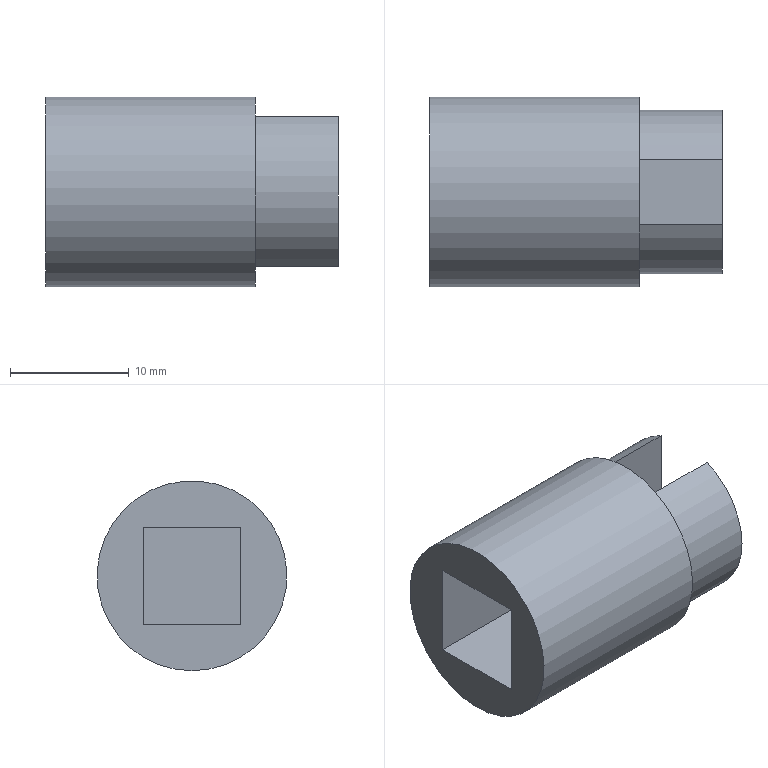Component | NX | SELECTOR_BLOCK | 1 solid | 17 faces | box 24.7 x 16 x 16 mm | volume 3205 mm3 | plane 14 | cylinder 3 | commonest cylinder face diameters 13.8 x2 16 x1
STEP:
#1=CARTESIAN_POINT('',(0.,0.,0.));
#2=DIRECTION('',(0.,0.,1.));
#3=DIRECTION('',(1.,0.,0.));
#4=AXIS2_PLACEMENT_3D('',#1,#2,#3);
#5=CARTESIAN_POINT('',(-16.538,-1.149,-12.417));
#6=VERTEX_POINT('',#5);
#7=CARTESIAN_POINT('',(-16.538,4.351,-12.417));
#8=VERTEX_POINT('',#7);
#9=CARTESIAN_POINT('',(-16.538,-1.149,-12.417));
#10=DIRECTION('',(0.,1.,-0.));
#11=VECTOR('',#10,1.);
#12=LINE('',#9,#11);
#13=CARTESIAN_POINT('',(-16.538,1.601,-11.667));
#14=DIRECTION('',(1.,0.,0.));
#15=DIRECTION('',(0.,0.,-1.));
#16=AXIS2_PLACEMENT_3D('',#13,#14,#15);
#17=PLANE('',#16);
#18=CARTESIAN_POINT('',(0.75,-2.75));
#19=DIRECTION('',(0.,1.));
#20=VECTOR('',#19,1.);
#21=LINE('',#18,#20);
#22=(GEOMETRIC_REPRESENTATION_CONTEXT(2)PARAMETRIC_REPRESENTATION_CONTEXT()REPRESENTATION_CONTEXT('',''));
#23=DEFINITIONAL_REPRESENTATION('',(#21),#22);
#24=PCURVE('',#17,#23);
#25=CARTESIAN_POINT('',(-23.538,-1.149,-12.417));
#26=DIRECTION('',(0.,-0.,-1.));
#27=DIRECTION('',(0.,1.,-0.));
#28=AXIS2_PLACEMENT_3D('',#25,#26,#27);
#29=PLANE('',#28);
#30=CARTESIAN_POINT('',(0.,7.));
#31=DIRECTION('',(1.,0.));
#32=VECTOR('',#31,1.);
#33=LINE('',#30,#32);
#34=(GEOMETRIC_REPRESENTATION_CONTEXT(2)PARAMETRIC_REPRESENTATION_CONTEXT()REPRESENTATION_CONTEXT('',''));
#35=DEFINITIONAL_REPRESENTATION('',(#33),#34);
#36=PCURVE('',#29,#35);
#37=SURFACE_CURVE('',#12,(#24,#36),.PCURVE_S1.);
#38=EDGE_CURVE('',#6,#8,#37,.T.);
#39=ORIENTED_EDGE('',*,*,#38,.T.);
#40=CARTESIAN_POINT('',(-16.538,4.351,-17.995));
#41=VERTEX_POINT('',#40);
#42=CARTESIAN_POINT('',(-16.538,4.351,-12.417));
#43=DIRECTION('',(0.,0.,-1.));
#44=VECTOR('',#43,1.);
#45=LINE('',#42,#44);
#46=CARTESIAN_POINT('',(0.75,2.75));
#47=DIRECTION('',(1.,0.));
#48=VECTOR('',#47,1.);
#49=LINE('',#46,#48);
#50=(GEOMETRIC_REPRESENTATION_CONTEXT(2)PARAMETRIC_REPRESENTATION_CONTEXT()REPRESENTATION_CONTEXT('',''));
#51=DEFINITIONAL_REPRESENTATION('',(#49),#50);
#52=PCURVE('',#17,#51);
#53=CARTESIAN_POINT('',(-23.538,4.351,-12.417));
#54=DIRECTION('',(0.,-1.,0.));
#55=DIRECTION('',(-1.,0.,0.));
#56=AXIS2_PLACEMENT_3D('',#53,#54,#55);
#57=PLANE('',#56);
#58=CARTESIAN_POINT('',(-7.,0.));
#59=DIRECTION('',(0.,1.));
#60=VECTOR('',#59,1.);
#61=LINE('',#58,#60);
#62=(GEOMETRIC_REPRESENTATION_CONTEXT(2)PARAMETRIC_REPRESENTATION_CONTEXT()REPRESENTATION_CONTEXT('',''));
#63=DEFINITIONAL_REPRESENTATION('',(#61),#62);
#64=PCURVE('',#57,#63);
#65=SURFACE_CURVE('',#45,(#52,#64),.PCURVE_S1.);
#66=EDGE_CURVE('',#8,#41,#65,.T.);
#67=ORIENTED_EDGE('',*,*,#66,.T.);
#68=CARTESIAN_POINT('',(-16.538,4.351,-5.338));
#69=VERTEX_POINT('',#68);
#70=CARTESIAN_POINT('',(-16.538,1.601,-11.667));
#71=DIRECTION('',(-1.,0.,0.));
#72=DIRECTION('',(0.,0.,-1.));
#73=AXIS2_PLACEMENT_3D('',#70,#71,#72);
#74=CIRCLE('',#73,6.9);
#75=CARTESIAN_POINT('',(6.9,0.));
#76=CARTESIAN_POINT('',(6.9,-11.951));
#77=CARTESIAN_POINT('',(-3.45,-5.976));
#78=CARTESIAN_POINT('',(-13.8,-0.));
#79=CARTESIAN_POINT('',(-3.45,5.976));
#80=CARTESIAN_POINT('',(6.9,11.951));
#81=CARTESIAN_POINT('',(6.9,0.));
#82=(BOUNDED_CURVE()B_SPLINE_CURVE(2,(#75,#76,#77,#78,#79,#80,#81),.UNSPECIFIED.,.T.,.F.)B_SPLINE_CURVE_WITH_KNOTS((1,2,2,2,2,1),(-2.094,0.,2.094,4.189,6.283,8.378),.UNSPECIFIED.)CURVE()GEOMETRIC_REPRESENTATION_ITEM()RATIONAL_B_SPLINE_CURVE((1.,0.5,1.,0.5,1.,0.5,1.))REPRESENTATION_ITEM(''));
#83=(GEOMETRIC_REPRESENTATION_CONTEXT(2)PARAMETRIC_REPRESENTATION_CONTEXT()REPRESENTATION_CONTEXT('',''));
#84=DEFINITIONAL_REPRESENTATION('',(#82),#83);
#85=PCURVE('',#17,#84);
#86=CARTESIAN_POINT('',(-23.538,1.601,-11.667));
#87=DIRECTION('',(1.,0.,0.));
#88=DIRECTION('',(0.,0.,-1.));
#89=AXIS2_PLACEMENT_3D('',#86,#87,#88);
#90=CYLINDRICAL_SURFACE('',#89,6.9);
#91=CARTESIAN_POINT('',(6.283,7.));
#92=DIRECTION('',(-1.,0.));
#93=VECTOR('',#92,1.);
#94=LINE('',#91,#93);
#95=(GEOMETRIC_REPRESENTATION_CONTEXT(2)PARAMETRIC_REPRESENTATION_CONTEXT()REPRESENTATION_CONTEXT('',''));
#96=DEFINITIONAL_REPRESENTATION('',(#94),#95);
#97=PCURVE('',#90,#96);
#98=SURFACE_CURVE('',#74,(#85,#97),.PCURVE_S1.);
#99=EDGE_CURVE('',#69,#41,#98,.T.);
#100=ORIENTED_EDGE('',*,*,#99,.F.);
#101=CARTESIAN_POINT('',(-16.538,4.351,-10.917));
#102=VERTEX_POINT('',#101);
#103=CARTESIAN_POINT('',(-16.538,4.351,-10.917));
#104=DIRECTION('',(0.,0.,1.));
#105=VECTOR('',#104,1.);
#106=LINE('',#103,#105);
#107=CARTESIAN_POINT('',(-0.75,2.75));
#108=DIRECTION('',(-1.,0.));
#109=VECTOR('',#108,1.);
#110=LINE('',#107,#109);
#111=(GEOMETRIC_REPRESENTATION_CONTEXT(2)PARAMETRIC_REPRESENTATION_CONTEXT()REPRESENTATION_CONTEXT('',''));
#112=DEFINITIONAL_REPRESENTATION('',(#110),#111);
#113=PCURVE('',#17,#112);
#114=CARTESIAN_POINT('',(-23.538,4.351,-10.917));
#115=DIRECTION('',(0.,1.,0.));
#116=DIRECTION('',(1.,0.,0.));
#117=AXIS2_PLACEMENT_3D('',#114,#115,#116);
#118=PLANE('',#117);
#119=CARTESIAN_POINT('',(7.,0.));
#120=DIRECTION('',(0.,-1.));
#121=VECTOR('',#120,1.);
#122=LINE('',#119,#121);
#123=(GEOMETRIC_REPRESENTATION_CONTEXT(2)PARAMETRIC_REPRESENTATION_CONTEXT()REPRESENTATION_CONTEXT('',''));
#124=DEFINITIONAL_REPRESENTATION('',(#122),#123);
#125=PCURVE('',#118,#124);
#126=SURFACE_CURVE('',#106,(#113,#125),.PCURVE_S1.);
#127=EDGE_CURVE('',#102,#69,#126,.T.);
#128=ORIENTED_EDGE('',*,*,#127,.F.);
#129=CARTESIAN_POINT('',(-16.538,-1.149,-10.917));
#130=VERTEX_POINT('',#129);
#131=CARTESIAN_POINT('',(-16.538,-1.149,-10.917));
#132=DIRECTION('',(0.,1.,0.));
#133=VECTOR('',#132,1.);
#134=LINE('',#131,#133);
#135=CARTESIAN_POINT('',(-0.75,-2.75));
#136=DIRECTION('',(-0.,1.));
#137=VECTOR('',#136,1.);
#138=LINE('',#135,#137);
#139=(GEOMETRIC_REPRESENTATION_CONTEXT(2)PARAMETRIC_REPRESENTATION_CONTEXT()REPRESENTATION_CONTEXT('',''));
#140=DEFINITIONAL_REPRESENTATION('',(#138),#139);
#141=PCURVE('',#17,#140);
#142=CARTESIAN_POINT('',(-23.538,-1.149,-10.917));
#143=DIRECTION('',(0.,0.,-1.));
#144=DIRECTION('',(0.,1.,0.));
#145=AXIS2_PLACEMENT_3D('',#142,#143,#144);
#146=PLANE('',#145);
#147=CARTESIAN_POINT('',(0.,7.));
#148=DIRECTION('',(1.,0.));
#149=VECTOR('',#148,1.);
#150=LINE('',#147,#149);
#151=(GEOMETRIC_REPRESENTATION_CONTEXT(2)PARAMETRIC_REPRESENTATION_CONTEXT()REPRESENTATION_CONTEXT('',''));
#152=DEFINITIONAL_REPRESENTATION('',(#150),#151);
#153=PCURVE('',#146,#152);
#154=SURFACE_CURVE('',#134,(#141,#153),.PCURVE_S1.);
#155=EDGE_CURVE('',#130,#102,#154,.T.);
#156=ORIENTED_EDGE('',*,*,#155,.F.);
#157=CARTESIAN_POINT('',(-16.538,-1.149,-5.338));
#158=VERTEX_POINT('',#157);
#159=CARTESIAN_POINT('',(-16.538,-1.149,1.183));
#160=DIRECTION('',(0.,0.,-1.));
#161=VECTOR('',#160,1.);
#162=LINE('',#159,#161);
#163=CARTESIAN_POINT('',(-12.85,-2.75));
#164=DIRECTION('',(1.,0.));
#165=VECTOR('',#164,1.);
#166=LINE('',#163,#165);
#167=(GEOMETRIC_REPRESENTATION_CONTEXT(2)PARAMETRIC_REPRESENTATION_CONTEXT()REPRESENTATION_CONTEXT('',''));
#168=DEFINITIONAL_REPRESENTATION('',(#166),#167);
#169=PCURVE('',#17,#168);
#170=CARTESIAN_POINT('',(-23.538,-1.149,1.183));
#171=DIRECTION('',(0.,-1.,-0.));
#172=DIRECTION('',(0.,0.,-1.));
#173=AXIS2_PLACEMENT_3D('',#170,#171,#172);
#174=PLANE('',#173);
#175=CARTESIAN_POINT('',(0.,7.));
#176=DIRECTION('',(1.,0.));
#177=VECTOR('',#176,1.);
#178=LINE('',#175,#177);
#179=(GEOMETRIC_REPRESENTATION_CONTEXT(2)PARAMETRIC_REPRESENTATION_CONTEXT()REPRESENTATION_CONTEXT('',''));
#180=DEFINITIONAL_REPRESENTATION('',(#178),#179);
#181=PCURVE('',#174,#180);
#182=SURFACE_CURVE('',#162,(#169,#181),.PCURVE_S1.);
#183=EDGE_CURVE('',#158,#130,#182,.T.);
#184=ORIENTED_EDGE('',*,*,#183,.F.);
#185=CARTESIAN_POINT('',(-16.538,-1.149,-17.995));
#186=VERTEX_POINT('',#185);
#187=CARTESIAN_POINT('',(-16.538,1.601,-11.667));
#188=DIRECTION('',(-1.,0.,0.));
#189=DIRECTION('',(0.,0.,-1.));
#190=AXIS2_PLACEMENT_3D('',#187,#188,#189);
#191=CIRCLE('',#190,6.9);
#192=CARTESIAN_POINT('',(6.9,0.));
#193=CARTESIAN_POINT('',(6.9,-11.951));
#194=CARTESIAN_POINT('',(-3.45,-5.976));
#195=CARTESIAN_POINT('',(-13.8,-0.));
#196=CARTESIAN_POINT('',(-3.45,5.976));
#197=CARTESIAN_POINT('',(6.9,11.951));
#198=CARTESIAN_POINT('',(6.9,0.));
#199=(BOUNDED_CURVE()B_SPLINE_CURVE(2,(#192,#193,#194,#195,#196,#197,#198),.UNSPECIFIED.,.T.,.F.)B_SPLINE_CURVE_WITH_KNOTS((1,2,2,2,2,1),(-2.094,0.,2.094,4.189,6.283,8.378),.UNSPECIFIED.)CURVE()GEOMETRIC_REPRESENTATION_ITEM()RATIONAL_B_SPLINE_CURVE((1.,0.5,1.,0.5,1.,0.5,1.))REPRESENTATION_ITEM(''));
#200=(GEOMETRIC_REPRESENTATION_CONTEXT(2)PARAMETRIC_REPRESENTATION_CONTEXT()REPRESENTATION_CONTEXT('',''));
#201=DEFINITIONAL_REPRESENTATION('',(#199),#200);
#202=PCURVE('',#17,#201);
#203=CARTESIAN_POINT('',(-23.538,1.601,-11.667));
#204=DIRECTION('',(1.,0.,0.));
#205=DIRECTION('',(0.,0.,-1.));
#206=AXIS2_PLACEMENT_3D('',#203,#204,#205);
#207=CYLINDRICAL_SURFACE('',#206,6.9);
#208=CARTESIAN_POINT('',(6.283,7.));
#209=DIRECTION('',(-1.,0.));
#210=VECTOR('',#209,1.);
#211=LINE('',#208,#210);
#212=(GEOMETRIC_REPRESENTATION_CONTEXT(2)PARAMETRIC_REPRESENTATION_CONTEXT()REPRESENTATION_CONTEXT('',''));
#213=DEFINITIONAL_REPRESENTATION('',(#211),#212);
#214=PCURVE('',#207,#213);
#215=SURFACE_CURVE('',#191,(#202,#214),.PCURVE_S1.);
#216=EDGE_CURVE('',#186,#158,#215,.T.);
#217=ORIENTED_EDGE('',*,*,#216,.F.);
#218=CARTESIAN_POINT('',(-16.538,-1.149,-24.517));
#219=DIRECTION('',(0.,0.,1.));
#220=VECTOR('',#219,1.);
#221=LINE('',#218,#220);
#222=CARTESIAN_POINT('',(12.85,-2.75));
#223=DIRECTION('',(-1.,0.));
#224=VECTOR('',#223,1.);
#225=LINE('',#222,#224);
#226=(GEOMETRIC_REPRESENTATION_CONTEXT(2)PARAMETRIC_REPRESENTATION_CONTEXT()REPRESENTATION_CONTEXT('',''));
#227=DEFINITIONAL_REPRESENTATION('',(#225),#226);
#228=PCURVE('',#17,#227);
#229=CARTESIAN_POINT('',(-23.538,-1.149,-24.517));
#230=DIRECTION('',(0.,1.,-0.));
#231=DIRECTION('',(0.,0.,1.));
#232=AXIS2_PLACEMENT_3D('',#229,#230,#231);
#233=PLANE('',#232);
#234=CARTESIAN_POINT('',(0.,7.));
#235=DIRECTION('',(1.,0.));
#236=VECTOR('',#235,1.);
#237=LINE('',#234,#236);
#238=(GEOMETRIC_REPRESENTATION_CONTEXT(2)PARAMETRIC_REPRESENTATION_CONTEXT()REPRESENTATION_CONTEXT('',''));
#239=DEFINITIONAL_REPRESENTATION('',(#237),#238);
#240=PCURVE('',#233,#239);
#241=SURFACE_CURVE('',#221,(#228,#240),.PCURVE_S1.);
#242=EDGE_CURVE('',#186,#6,#241,.T.);
#243=ORIENTED_EDGE('',*,*,#242,.T.);
#244=EDGE_LOOP('',(#39,#67,#100,#128,#156,#184,#217,#243));
#245=FACE_BOUND('',#244,.T.);
#246=ADVANCED_FACE('',(#245),#17,.T.);
#247=CARTESIAN_POINT('',(-23.538,-1.149,-5.338));
#248=VERTEX_POINT('',#247);
#249=CARTESIAN_POINT('',(-23.538,-1.149,-17.995));
#250=VERTEX_POINT('',#249);
#251=CARTESIAN_POINT('',(-23.538,1.601,-11.667));
#252=DIRECTION('',(1.,0.,0.));
#253=DIRECTION('',(0.,0.,-1.));
#254=AXIS2_PLACEMENT_3D('',#251,#252,#253);
#255=CIRCLE('',#254,6.9);
#256=CARTESIAN_POINT('',(-0.,0.));
#257=DIRECTION('',(1.,0.));
#258=VECTOR('',#257,1.);
#259=LINE('',#256,#258);
#260=(GEOMETRIC_REPRESENTATION_CONTEXT(2)PARAMETRIC_REPRESENTATION_CONTEXT()REPRESENTATION_CONTEXT('',''));
#261=DEFINITIONAL_REPRESENTATION('',(#259),#260);
#262=PCURVE('',#207,#261);
#263=CARTESIAN_POINT('',(-23.538,1.601,-11.667));
#264=DIRECTION('',(1.,0.,0.));
#265=DIRECTION('',(0.,0.,-1.));
#266=AXIS2_PLACEMENT_3D('',#263,#264,#265);
#267=PLANE('',#266);
#268=CARTESIAN_POINT('',(0.,0.));
#269=DIRECTION('',(1.,0.));
#270=AXIS2_PLACEMENT_2D('',#268,#269);
#271=CIRCLE('',#270,6.9);
#272=(GEOMETRIC_REPRESENTATION_CONTEXT(2)PARAMETRIC_REPRESENTATION_CONTEXT()REPRESENTATION_CONTEXT('',''));
#273=DEFINITIONAL_REPRESENTATION('',(#271),#272);
#274=PCURVE('',#267,#273);
#275=SURFACE_CURVE('',#255,(#262,#274),.PCURVE_S1.);
#276=EDGE_CURVE('',#248,#250,#275,.T.);
#277=ORIENTED_EDGE('',*,*,#276,.T.);
#278=CARTESIAN_POINT('',(-23.538,-1.149,-17.995));
#279=DIRECTION('',(1.,0.,0.));
#280=VECTOR('',#279,1.);
#281=LINE('',#278,#280);
#282=CARTESIAN_POINT('',(5.873,0.));
#283=DIRECTION('',(0.,1.));
#284=VECTOR('',#283,1.);
#285=LINE('',#282,#284);
#286=(GEOMETRIC_REPRESENTATION_CONTEXT(2)PARAMETRIC_REPRESENTATION_CONTEXT()REPRESENTATION_CONTEXT('',''));
#287=DEFINITIONAL_REPRESENTATION('',(#285),#286);
#288=PCURVE('',#207,#287);
#289=CARTESIAN_POINT('',(6.522,0.));
#290=DIRECTION('',(0.,1.));
#291=VECTOR('',#290,1.);
#292=LINE('',#289,#291);
#293=(GEOMETRIC_REPRESENTATION_CONTEXT(2)PARAMETRIC_REPRESENTATION_CONTEXT()REPRESENTATION_CONTEXT('',''));
#294=DEFINITIONAL_REPRESENTATION('',(#292),#293);
#295=PCURVE('',#233,#294);
#296=SURFACE_CURVE('',#281,(#288,#295),.PCURVE_S1.);
#297=EDGE_CURVE('',#250,#186,#296,.T.);
#298=ORIENTED_EDGE('',*,*,#297,.T.);
#299=ORIENTED_EDGE('',*,*,#216,.T.);
#300=CARTESIAN_POINT('',(-23.538,-1.149,-5.338));
#301=DIRECTION('',(1.,0.,0.));
#302=VECTOR('',#301,1.);
#303=LINE('',#300,#302);
#304=CARTESIAN_POINT('',(3.552,0.));
#305=DIRECTION('',(0.,1.));
#306=VECTOR('',#305,1.);
#307=LINE('',#304,#306);
#308=(GEOMETRIC_REPRESENTATION_CONTEXT(2)PARAMETRIC_REPRESENTATION_CONTEXT()REPRESENTATION_CONTEXT('',''));
#309=DEFINITIONAL_REPRESENTATION('',(#307),#308);
#310=PCURVE('',#207,#309);
#311=CARTESIAN_POINT('',(6.522,0.));
#312=DIRECTION('',(0.,1.));
#313=VECTOR('',#312,1.);
#314=LINE('',#311,#313);
#315=(GEOMETRIC_REPRESENTATION_CONTEXT(2)PARAMETRIC_REPRESENTATION_CONTEXT()REPRESENTATION_CONTEXT('',''));
#316=DEFINITIONAL_REPRESENTATION('',(#314),#315);
#317=PCURVE('',#174,#316);
#318=SURFACE_CURVE('',#303,(#310,#317),.PCURVE_S1.);
#319=EDGE_CURVE('',#248,#158,#318,.T.);
#320=ORIENTED_EDGE('',*,*,#319,.F.);
#321=EDGE_LOOP('',(#277,#298,#299,#320));
#322=FACE_BOUND('',#321,.T.);
#323=ADVANCED_FACE('',(#322),#207,.T.);
#324=ORIENTED_EDGE('',*,*,#99,.T.);
#325=CARTESIAN_POINT('',(-23.538,4.351,-17.995));
#326=VERTEX_POINT('',#325);
#327=CARTESIAN_POINT('',(-23.538,4.351,-17.995));
#328=DIRECTION('',(-1.,0.,0.));
#329=VECTOR('',#328,1.);
#330=LINE('',#327,#329);
#331=CARTESIAN_POINT('',(0.4099,0.));
#332=DIRECTION('',(0.,-1.));
#333=VECTOR('',#332,1.);
#334=LINE('',#331,#333);
#335=(GEOMETRIC_REPRESENTATION_CONTEXT(2)PARAMETRIC_REPRESENTATION_CONTEXT()REPRESENTATION_CONTEXT('',''));
#336=DEFINITIONAL_REPRESENTATION('',(#334),#335);
#337=PCURVE('',#90,#336);
#338=CARTESIAN_POINT('',(0.,5.578));
#339=DIRECTION('',(1.,0.));
#340=VECTOR('',#339,1.);
#341=LINE('',#338,#340);
#342=(GEOMETRIC_REPRESENTATION_CONTEXT(2)PARAMETRIC_REPRESENTATION_CONTEXT()REPRESENTATION_CONTEXT('',''));
#343=DEFINITIONAL_REPRESENTATION('',(#341),#342);
#344=PCURVE('',#57,#343);
#345=SURFACE_CURVE('',#330,(#337,#344),.PCURVE_S1.);
#346=EDGE_CURVE('',#41,#326,#345,.T.);
#347=ORIENTED_EDGE('',*,*,#346,.T.);
#348=CARTESIAN_POINT('',(-23.538,4.351,-5.338));
#349=VERTEX_POINT('',#348);
#350=CARTESIAN_POINT('',(-23.538,1.601,-11.667));
#351=DIRECTION('',(1.,0.,0.));
#352=DIRECTION('',(0.,0.,-1.));
#353=AXIS2_PLACEMENT_3D('',#350,#351,#352);
#354=CIRCLE('',#353,6.9);
#355=CARTESIAN_POINT('',(0.,0.));
#356=DIRECTION('',(1.,0.));
#357=VECTOR('',#356,1.);
#358=LINE('',#355,#357);
#359=(GEOMETRIC_REPRESENTATION_CONTEXT(2)PARAMETRIC_REPRESENTATION_CONTEXT()REPRESENTATION_CONTEXT('',''));
#360=DEFINITIONAL_REPRESENTATION('',(#358),#359);
#361=PCURVE('',#90,#360);
#362=CARTESIAN_POINT('',(0.,0.));
#363=DIRECTION('',(1.,0.));
#364=AXIS2_PLACEMENT_2D('',#362,#363);
#365=CIRCLE('',#364,6.9);
#366=(GEOMETRIC_REPRESENTATION_CONTEXT(2)PARAMETRIC_REPRESENTATION_CONTEXT()REPRESENTATION_CONTEXT('',''));
#367=DEFINITIONAL_REPRESENTATION('',(#365),#366);
#368=PCURVE('',#267,#367);
#369=SURFACE_CURVE('',#354,(#361,#368),.PCURVE_S1.);
#370=EDGE_CURVE('',#326,#349,#369,.T.);
#371=ORIENTED_EDGE('',*,*,#370,.T.);
#372=CARTESIAN_POINT('',(-23.538,4.351,-5.338));
#373=DIRECTION('',(-1.,0.,0.));
#374=VECTOR('',#373,1.);
#375=LINE('',#372,#374);
#376=CARTESIAN_POINT('',(2.732,0.));
#377=DIRECTION('',(0.,-1.));
#378=VECTOR('',#377,1.);
#379=LINE('',#376,#378);
#380=(GEOMETRIC_REPRESENTATION_CONTEXT(2)PARAMETRIC_REPRESENTATION_CONTEXT()REPRESENTATION_CONTEXT('',''));
#381=DEFINITIONAL_REPRESENTATION('',(#379),#380);
#382=PCURVE('',#90,#381);
#383=CARTESIAN_POINT('',(0.,-5.578));
#384=DIRECTION('',(-1.,0.));
#385=VECTOR('',#384,1.);
#386=LINE('',#383,#385);
#387=(GEOMETRIC_REPRESENTATION_CONTEXT(2)PARAMETRIC_REPRESENTATION_CONTEXT()REPRESENTATION_CONTEXT('',''));
#388=DEFINITIONAL_REPRESENTATION('',(#386),#387);
#389=PCURVE('',#118,#388);
#390=SURFACE_CURVE('',#375,(#382,#389),.PCURVE_S1.);
#391=EDGE_CURVE('',#69,#349,#390,.T.);
#392=ORIENTED_EDGE('',*,*,#391,.F.);
#393=EDGE_LOOP('',(#324,#347,#371,#392));
#394=FACE_BOUND('',#393,.T.);
#395=ADVANCED_FACE('',(#394),#90,.T.);
#396=ORIENTED_EDGE('',*,*,#370,.F.);
#397=CARTESIAN_POINT('',(-23.538,4.351,-12.417));
#398=VERTEX_POINT('',#397);
#399=CARTESIAN_POINT('',(-23.538,4.351,-12.417));
#400=DIRECTION('',(0.,0.,-1.));
#401=VECTOR('',#400,1.);
#402=LINE('',#399,#401);
#403=CARTESIAN_POINT('',(0.75,2.75));
#404=DIRECTION('',(1.,0.));
#405=VECTOR('',#404,1.);
#406=LINE('',#403,#405);
#407=(GEOMETRIC_REPRESENTATION_CONTEXT(2)PARAMETRIC_REPRESENTATION_CONTEXT()REPRESENTATION_CONTEXT('',''));
#408=DEFINITIONAL_REPRESENTATION('',(#406),#407);
#409=PCURVE('',#267,#408);
#410=CARTESIAN_POINT('',(0.,0.));
#411=DIRECTION('',(0.,1.));
#412=VECTOR('',#411,1.);
#413=LINE('',#410,#412);
#414=(GEOMETRIC_REPRESENTATION_CONTEXT(2)PARAMETRIC_REPRESENTATION_CONTEXT()REPRESENTATION_CONTEXT('',''));
#415=DEFINITIONAL_REPRESENTATION('',(#413),#414);
#416=PCURVE('',#57,#415);
#417=SURFACE_CURVE('',#402,(#409,#416),.PCURVE_S1.);
#418=EDGE_CURVE('',#398,#326,#417,.T.);
#419=ORIENTED_EDGE('',*,*,#418,.F.);
#420=CARTESIAN_POINT('',(-23.538,-1.149,-12.417));
#421=VERTEX_POINT('',#420);
#422=CARTESIAN_POINT('',(-23.538,-1.149,-12.417));
#423=DIRECTION('',(0.,1.,-0.));
#424=VECTOR('',#423,1.);
#425=LINE('',#422,#424);
#426=CARTESIAN_POINT('',(0.75,-2.75));
#427=DIRECTION('',(0.,1.));
#428=VECTOR('',#427,1.);
#429=LINE('',#426,#428);
#430=(GEOMETRIC_REPRESENTATION_CONTEXT(2)PARAMETRIC_REPRESENTATION_CONTEXT()REPRESENTATION_CONTEXT('',''));
#431=DEFINITIONAL_REPRESENTATION('',(#429),#430);
#432=PCURVE('',#267,#431);
#433=CARTESIAN_POINT('',(0.,0.));
#434=DIRECTION('',(1.,0.));
#435=VECTOR('',#434,1.);
#436=LINE('',#433,#435);
#437=(GEOMETRIC_REPRESENTATION_CONTEXT(2)PARAMETRIC_REPRESENTATION_CONTEXT()REPRESENTATION_CONTEXT('',''));
#438=DEFINITIONAL_REPRESENTATION('',(#436),#437);
#439=PCURVE('',#29,#438);
#440=SURFACE_CURVE('',#425,(#432,#439),.PCURVE_S1.);
#441=EDGE_CURVE('',#421,#398,#440,.T.);
#442=ORIENTED_EDGE('',*,*,#441,.F.);
#443=CARTESIAN_POINT('',(-23.538,-1.149,-24.517));
#444=DIRECTION('',(0.,0.,1.));
#445=VECTOR('',#444,1.);
#446=LINE('',#443,#445);
#447=CARTESIAN_POINT('',(12.85,-2.75));
#448=DIRECTION('',(-1.,0.));
#449=VECTOR('',#448,1.);
#450=LINE('',#447,#449);
#451=(GEOMETRIC_REPRESENTATION_CONTEXT(2)PARAMETRIC_REPRESENTATION_CONTEXT()REPRESENTATION_CONTEXT('',''));
#452=DEFINITIONAL_REPRESENTATION('',(#450),#451);
#453=PCURVE('',#267,#452);
#454=CARTESIAN_POINT('',(0.,0.));
#455=DIRECTION('',(1.,0.));
#456=VECTOR('',#455,1.);
#457=LINE('',#454,#456);
#458=(GEOMETRIC_REPRESENTATION_CONTEXT(2)PARAMETRIC_REPRESENTATION_CONTEXT()REPRESENTATION_CONTEXT('',''));
#459=DEFINITIONAL_REPRESENTATION('',(#457),#458);
#460=PCURVE('',#233,#459);
#461=SURFACE_CURVE('',#446,(#453,#460),.PCURVE_S1.);
#462=EDGE_CURVE('',#250,#421,#461,.T.);
#463=ORIENTED_EDGE('',*,*,#462,.F.);
#464=ORIENTED_EDGE('',*,*,#276,.F.);
#465=CARTESIAN_POINT('',(-23.538,-1.149,-10.917));
#466=VERTEX_POINT('',#465);
#467=CARTESIAN_POINT('',(-23.538,-1.149,1.183));
#468=DIRECTION('',(0.,0.,-1.));
#469=VECTOR('',#468,1.);
#470=LINE('',#467,#469);
#471=CARTESIAN_POINT('',(-12.85,-2.75));
#472=DIRECTION('',(1.,0.));
#473=VECTOR('',#472,1.);
#474=LINE('',#471,#473);
#475=(GEOMETRIC_REPRESENTATION_CONTEXT(2)PARAMETRIC_REPRESENTATION_CONTEXT()REPRESENTATION_CONTEXT('',''));
#476=DEFINITIONAL_REPRESENTATION('',(#474),#475);
#477=PCURVE('',#267,#476);
#478=CARTESIAN_POINT('',(0.,0.));
#479=DIRECTION('',(1.,0.));
#480=VECTOR('',#479,1.);
#481=LINE('',#478,#480);
#482=(GEOMETRIC_REPRESENTATION_CONTEXT(2)PARAMETRIC_REPRESENTATION_CONTEXT()REPRESENTATION_CONTEXT('',''));
#483=DEFINITIONAL_REPRESENTATION('',(#481),#482);
#484=PCURVE('',#174,#483);
#485=SURFACE_CURVE('',#470,(#477,#484),.PCURVE_S1.);
#486=EDGE_CURVE('',#248,#466,#485,.T.);
#487=ORIENTED_EDGE('',*,*,#486,.T.);
#488=CARTESIAN_POINT('',(-23.538,4.351,-10.917));
#489=VERTEX_POINT('',#488);
#490=CARTESIAN_POINT('',(-23.538,-1.149,-10.917));
#491=DIRECTION('',(0.,1.,0.));
#492=VECTOR('',#491,1.);
#493=LINE('',#490,#492);
#494=CARTESIAN_POINT('',(-0.75,-2.75));
#495=DIRECTION('',(-0.,1.));
#496=VECTOR('',#495,1.);
#497=LINE('',#494,#496);
#498=(GEOMETRIC_REPRESENTATION_CONTEXT(2)PARAMETRIC_REPRESENTATION_CONTEXT()REPRESENTATION_CONTEXT('',''));
#499=DEFINITIONAL_REPRESENTATION('',(#497),#498);
#500=PCURVE('',#267,#499);
#501=CARTESIAN_POINT('',(0.,0.));
#502=DIRECTION('',(1.,0.));
#503=VECTOR('',#502,1.);
#504=LINE('',#501,#503);
#505=(GEOMETRIC_REPRESENTATION_CONTEXT(2)PARAMETRIC_REPRESENTATION_CONTEXT()REPRESENTATION_CONTEXT('',''));
#506=DEFINITIONAL_REPRESENTATION('',(#504),#505);
#507=PCURVE('',#146,#506);
#508=SURFACE_CURVE('',#493,(#500,#507),.PCURVE_S1.);
#509=EDGE_CURVE('',#466,#489,#508,.T.);
#510=ORIENTED_EDGE('',*,*,#509,.T.);
#511=CARTESIAN_POINT('',(-23.538,4.351,-10.917));
#512=DIRECTION('',(0.,0.,1.));
#513=VECTOR('',#512,1.);
#514=LINE('',#511,#513);
#515=CARTESIAN_POINT('',(-0.75,2.75));
#516=DIRECTION('',(-1.,0.));
#517=VECTOR('',#516,1.);
#518=LINE('',#515,#517);
#519=(GEOMETRIC_REPRESENTATION_CONTEXT(2)PARAMETRIC_REPRESENTATION_CONTEXT()REPRESENTATION_CONTEXT('',''));
#520=DEFINITIONAL_REPRESENTATION('',(#518),#519);
#521=PCURVE('',#267,#520);
#522=CARTESIAN_POINT('',(0.,0.));
#523=DIRECTION('',(0.,-1.));
#524=VECTOR('',#523,1.);
#525=LINE('',#522,#524);
#526=(GEOMETRIC_REPRESENTATION_CONTEXT(2)PARAMETRIC_REPRESENTATION_CONTEXT()REPRESENTATION_CONTEXT('',''));
#527=DEFINITIONAL_REPRESENTATION('',(#525),#526);
#528=PCURVE('',#118,#527);
#529=SURFACE_CURVE('',#514,(#521,#528),.PCURVE_S1.);
#530=EDGE_CURVE('',#489,#349,#529,.T.);
#531=ORIENTED_EDGE('',*,*,#530,.T.);
#532=EDGE_LOOP('',(#396,#419,#442,#463,#464,#487,#510,#531));
#533=FACE_BOUND('',#532,.T.);
#534=CARTESIAN_POINT('',(-23.538,1.601,-19.667));
#535=VERTEX_POINT('',#534);
#536=CARTESIAN_POINT('',(-23.538,1.601,-11.667));
#537=DIRECTION('',(-1.,0.,0.));
#538=DIRECTION('',(0.,0.,-1.));
#539=AXIS2_PLACEMENT_3D('',#536,#537,#538);
#540=CIRCLE('',#539,8.);
#541=CARTESIAN_POINT('',(8.,0.));
#542=CARTESIAN_POINT('',(8.,-13.856));
#543=CARTESIAN_POINT('',(-4.,-6.928));
#544=CARTESIAN_POINT('',(-16.,-0.));
#545=CARTESIAN_POINT('',(-4.,6.928));
#546=CARTESIAN_POINT('',(8.,13.856));
#547=CARTESIAN_POINT('',(8.,0.));
#548=(BOUNDED_CURVE()B_SPLINE_CURVE(2,(#541,#542,#543,#544,#545,#546,#547),.UNSPECIFIED.,.T.,.F.)B_SPLINE_CURVE_WITH_KNOTS((1,2,2,2,2,1),(-2.094,0.,2.094,4.189,6.283,8.378),.UNSPECIFIED.)CURVE()GEOMETRIC_REPRESENTATION_ITEM()RATIONAL_B_SPLINE_CURVE((1.,0.5,1.,0.5,1.,0.5,1.))REPRESENTATION_ITEM(''));
#549=(GEOMETRIC_REPRESENTATION_CONTEXT(2)PARAMETRIC_REPRESENTATION_CONTEXT()REPRESENTATION_CONTEXT('',''));
#550=DEFINITIONAL_REPRESENTATION('',(#548),#549);
#551=PCURVE('',#267,#550);
#552=CARTESIAN_POINT('',(-41.238,1.601,-11.667));
#553=DIRECTION('',(1.,0.,0.));
#554=DIRECTION('',(0.,0.,-1.));
#555=AXIS2_PLACEMENT_3D('',#552,#553,#554);
#556=CYLINDRICAL_SURFACE('',#555,8.);
#557=CARTESIAN_POINT('',(6.283,17.7));
#558=DIRECTION('',(-1.,0.));
#559=VECTOR('',#558,1.);
#560=LINE('',#557,#559);
#561=(GEOMETRIC_REPRESENTATION_CONTEXT(2)PARAMETRIC_REPRESENTATION_CONTEXT()REPRESENTATION_CONTEXT('',''));
#562=DEFINITIONAL_REPRESENTATION('',(#560),#561);
#563=PCURVE('',#556,#562);
#564=SURFACE_CURVE('',#540,(#551,#563),.PCURVE_S1.);
#565=EDGE_CURVE('',#535,#535,#564,.T.);
#566=ORIENTED_EDGE('',*,*,#565,.F.);
#567=EDGE_LOOP('',(#566));
#568=FACE_BOUND('',#567,.T.);
#569=ADVANCED_FACE('',(#533,#568),#267,.T.);
#570=CARTESIAN_POINT('',(-41.238,-2.499,-7.567));
#571=VERTEX_POINT('',#570);
#572=CARTESIAN_POINT('',(-41.238,5.701,-7.567));
#573=VERTEX_POINT('',#572);
#574=CARTESIAN_POINT('',(-41.238,-2.499,-7.567));
#575=DIRECTION('',(0.,1.,0.));
#576=VECTOR('',#575,1.);
#577=LINE('',#574,#576);
#578=CARTESIAN_POINT('',(-41.238,1.601,-11.667));
#579=DIRECTION('',(-1.,0.,0.));
#580=DIRECTION('',(0.,0.,1.));
#581=AXIS2_PLACEMENT_3D('',#578,#579,#580);
#582=PLANE('',#581);
#583=CARTESIAN_POINT('',(4.1,-4.1));
#584=DIRECTION('',(0.,1.));
#585=VECTOR('',#584,1.);
#586=LINE('',#583,#585);
#587=(GEOMETRIC_REPRESENTATION_CONTEXT(2)PARAMETRIC_REPRESENTATION_CONTEXT()REPRESENTATION_CONTEXT('',''));
#588=DEFINITIONAL_REPRESENTATION('',(#586),#587);
#589=PCURVE('',#582,#588);
#590=CARTESIAN_POINT('',(-27.238,-2.499,-7.567));
#591=DIRECTION('',(0.,0.,1.));
#592=DIRECTION('',(1.,0.,0.));
#593=AXIS2_PLACEMENT_3D('',#590,#591,#592);
#594=PLANE('',#593);
#595=CARTESIAN_POINT('',(-14.,0.));
#596=DIRECTION('',(0.,1.));
#597=VECTOR('',#596,1.);
#598=LINE('',#595,#597);
#599=(GEOMETRIC_REPRESENTATION_CONTEXT(2)PARAMETRIC_REPRESENTATION_CONTEXT()REPRESENTATION_CONTEXT('',''));
#600=DEFINITIONAL_REPRESENTATION('',(#598),#599);
#601=PCURVE('',#594,#600);
#602=SURFACE_CURVE('',#577,(#589,#601),.PCURVE_S1.);
#603=EDGE_CURVE('',#571,#573,#602,.T.);
#604=ORIENTED_EDGE('',*,*,#603,.F.);
#605=CARTESIAN_POINT('',(-41.238,-2.499,-15.767));
#606=VERTEX_POINT('',#605);
#607=CARTESIAN_POINT('',(-41.238,-2.499,-15.767));
#608=DIRECTION('',(0.,0.,1.));
#609=VECTOR('',#608,1.);
#610=LINE('',#607,#609);
#611=CARTESIAN_POINT('',(-4.1,-4.1));
#612=DIRECTION('',(1.,0.));
#613=VECTOR('',#612,1.);
#614=LINE('',#611,#613);
#615=(GEOMETRIC_REPRESENTATION_CONTEXT(2)PARAMETRIC_REPRESENTATION_CONTEXT()REPRESENTATION_CONTEXT('',''));
#616=DEFINITIONAL_REPRESENTATION('',(#614),#615);
#617=PCURVE('',#582,#616);
#618=CARTESIAN_POINT('',(-27.238,-2.499,-15.767));
#619=DIRECTION('',(0.,-1.,0.));
#620=DIRECTION('',(-1.,0.,0.));
#621=AXIS2_PLACEMENT_3D('',#618,#619,#620);
#622=PLANE('',#621);
#623=CARTESIAN_POINT('',(14.,0.));
#624=DIRECTION('',(0.,-1.));
#625=VECTOR('',#624,1.);
#626=LINE('',#623,#625);
#627=(GEOMETRIC_REPRESENTATION_CONTEXT(2)PARAMETRIC_REPRESENTATION_CONTEXT()REPRESENTATION_CONTEXT('',''));
#628=DEFINITIONAL_REPRESENTATION('',(#626),#627);
#629=PCURVE('',#622,#628);
#630=SURFACE_CURVE('',#610,(#617,#629),.PCURVE_S1.);
#631=EDGE_CURVE('',#606,#571,#630,.T.);
#632=ORIENTED_EDGE('',*,*,#631,.F.);
#633=CARTESIAN_POINT('',(-41.238,5.701,-15.767));
#634=VERTEX_POINT('',#633);
#635=CARTESIAN_POINT('',(-41.238,5.701,-15.767));
#636=DIRECTION('',(0.,-1.,0.));
#637=VECTOR('',#636,1.);
#638=LINE('',#635,#637);
#639=CARTESIAN_POINT('',(-4.1,4.1));
#640=DIRECTION('',(0.,-1.));
#641=VECTOR('',#640,1.);
#642=LINE('',#639,#641);
#643=(GEOMETRIC_REPRESENTATION_CONTEXT(2)PARAMETRIC_REPRESENTATION_CONTEXT()REPRESENTATION_CONTEXT('',''));
#644=DEFINITIONAL_REPRESENTATION('',(#642),#643);
#645=PCURVE('',#582,#644);
#646=CARTESIAN_POINT('',(-27.238,5.701,-15.767));
#647=DIRECTION('',(0.,0.,-1.));
#648=DIRECTION('',(-1.,0.,0.));
#649=AXIS2_PLACEMENT_3D('',#646,#647,#648);
#650=PLANE('',#649);
#651=CARTESIAN_POINT('',(14.,0.));
#652=DIRECTION('',(0.,-1.));
#653=VECTOR('',#652,1.);
#654=LINE('',#651,#653);
#655=(GEOMETRIC_REPRESENTATION_CONTEXT(2)PARAMETRIC_REPRESENTATION_CONTEXT()REPRESENTATION_CONTEXT('',''));
#656=DEFINITIONAL_REPRESENTATION('',(#654),#655);
#657=PCURVE('',#650,#656);
#658=SURFACE_CURVE('',#638,(#645,#657),.PCURVE_S1.);
#659=EDGE_CURVE('',#634,#606,#658,.T.);
#660=ORIENTED_EDGE('',*,*,#659,.F.);
#661=CARTESIAN_POINT('',(-41.238,5.701,-7.567));
#662=DIRECTION('',(0.,0.,-1.));
#663=VECTOR('',#662,1.);
#664=LINE('',#661,#663);
#665=CARTESIAN_POINT('',(4.1,4.1));
#666=DIRECTION('',(-1.,0.));
#667=VECTOR('',#666,1.);
#668=LINE('',#665,#667);
#669=(GEOMETRIC_REPRESENTATION_CONTEXT(2)PARAMETRIC_REPRESENTATION_CONTEXT()REPRESENTATION_CONTEXT('',''));
#670=DEFINITIONAL_REPRESENTATION('',(#668),#669);
#671=PCURVE('',#582,#670);
#672=CARTESIAN_POINT('',(-27.238,5.701,-7.567));
#673=DIRECTION('',(0.,1.,0.));
#674=DIRECTION('',(1.,0.,0.));
#675=AXIS2_PLACEMENT_3D('',#672,#673,#674);
#676=PLANE('',#675);
#677=CARTESIAN_POINT('',(-14.,0.));
#678=DIRECTION('',(0.,1.));
#679=VECTOR('',#678,1.);
#680=LINE('',#677,#679);
#681=(GEOMETRIC_REPRESENTATION_CONTEXT(2)PARAMETRIC_REPRESENTATION_CONTEXT()REPRESENTATION_CONTEXT('',''));
#682=DEFINITIONAL_REPRESENTATION('',(#680),#681);
#683=PCURVE('',#676,#682);
#684=SURFACE_CURVE('',#664,(#671,#683),.PCURVE_S1.);
#685=EDGE_CURVE('',#573,#634,#684,.T.);
#686=ORIENTED_EDGE('',*,*,#685,.F.);
#687=EDGE_LOOP('',(#604,#632,#660,#686));
#688=FACE_BOUND('',#687,.T.);
#689=CARTESIAN_POINT('',(-41.238,1.601,-19.667));
#690=VERTEX_POINT('',#689);
#691=CARTESIAN_POINT('',(-41.238,1.601,-11.667));
#692=DIRECTION('',(1.,0.,0.));
#693=DIRECTION('',(0.,0.,-1.));
#694=AXIS2_PLACEMENT_3D('',#691,#692,#693);
#695=CIRCLE('',#694,8.);
#696=CARTESIAN_POINT('',(-8.,0.));
#697=CARTESIAN_POINT('',(-8.,13.856));
#698=CARTESIAN_POINT('',(4.,6.928));
#699=CARTESIAN_POINT('',(16.,0.));
#700=CARTESIAN_POINT('',(4.,-6.928));
#701=CARTESIAN_POINT('',(-8.,-13.856));
#702=CARTESIAN_POINT('',(-8.,0.));
#703=(BOUNDED_CURVE()B_SPLINE_CURVE(2,(#696,#697,#698,#699,#700,#701,#702),.UNSPECIFIED.,.T.,.F.)B_SPLINE_CURVE_WITH_KNOTS((1,2,2,2,2,1),(-2.094,0.,2.094,4.189,6.283,8.378),.UNSPECIFIED.)CURVE()GEOMETRIC_REPRESENTATION_ITEM()RATIONAL_B_SPLINE_CURVE((1.,0.5,1.,0.5,1.,0.5,1.))REPRESENTATION_ITEM(''));
#704=(GEOMETRIC_REPRESENTATION_CONTEXT(2)PARAMETRIC_REPRESENTATION_CONTEXT()REPRESENTATION_CONTEXT('',''));
#705=DEFINITIONAL_REPRESENTATION('',(#703),#704);
#706=PCURVE('',#582,#705);
#707=CARTESIAN_POINT('',(0.,0.));
#708=DIRECTION('',(1.,0.));
#709=VECTOR('',#708,1.);
#710=LINE('',#707,#709);
#711=(GEOMETRIC_REPRESENTATION_CONTEXT(2)PARAMETRIC_REPRESENTATION_CONTEXT()REPRESENTATION_CONTEXT('',''));
#712=DEFINITIONAL_REPRESENTATION('',(#710),#711);
#713=PCURVE('',#556,#712);
#714=SURFACE_CURVE('',#695,(#706,#713),.PCURVE_S1.);
#715=EDGE_CURVE('',#690,#690,#714,.T.);
#716=ORIENTED_EDGE('',*,*,#715,.F.);
#717=EDGE_LOOP('',(#716));
#718=FACE_BOUND('',#717,.T.);
#719=ADVANCED_FACE('',(#688,#718),#582,.T.);
#720=ORIENTED_EDGE('',*,*,#565,.T.);
#721=CARTESIAN_POINT('',(-41.238,1.601,-19.667));
#722=CARTESIAN_POINT('',(-23.538,1.601,-19.667));
#723=B_SPLINE_CURVE_WITH_KNOTS('',1,(#721,#722),.UNSPECIFIED.,.F.,.F.,(2,2),(0.,17.7),.PIECEWISE_BEZIER_KNOTS.);
#724=CARTESIAN_POINT('',(0.,0.));
#725=DIRECTION('',(0.,1.));
#726=VECTOR('',#725,1.);
#727=LINE('',#724,#726);
#728=(GEOMETRIC_REPRESENTATION_CONTEXT(2)PARAMETRIC_REPRESENTATION_CONTEXT()REPRESENTATION_CONTEXT('',''));
#729=DEFINITIONAL_REPRESENTATION('',(#727),#728);
#730=PCURVE('',#556,#729);
#731=CARTESIAN_POINT('',(6.283,0.));
#732=DIRECTION('',(0.,1.));
#733=VECTOR('',#732,1.);
#734=LINE('',#731,#733);
#735=(GEOMETRIC_REPRESENTATION_CONTEXT(2)PARAMETRIC_REPRESENTATION_CONTEXT()REPRESENTATION_CONTEXT('',''));
#736=DEFINITIONAL_REPRESENTATION('',(#734),#735);
#737=PCURVE('',#556,#736);
#738=SEAM_CURVE('',#723,(#730,#737),.PCURVE_S1.);
#739=EDGE_CURVE('',#690,#535,#738,.T.);
#740=ORIENTED_EDGE('',*,*,#739,.F.);
#741=ORIENTED_EDGE('',*,*,#715,.T.);
#742=ORIENTED_EDGE('',*,*,#739,.T.);
#743=EDGE_LOOP('',(#720,#740,#741,#742));
#744=FACE_BOUND('',#743,.T.);
#745=ADVANCED_FACE('',(#744),#556,.T.);
#746=ORIENTED_EDGE('',*,*,#319,.T.);
#747=ORIENTED_EDGE('',*,*,#183,.T.);
#748=CARTESIAN_POINT('',(-23.538,-1.149,-10.917));
#749=DIRECTION('',(-1.,0.,0.));
#750=VECTOR('',#749,1.);
#751=LINE('',#748,#750);
#752=CARTESIAN_POINT('',(12.1,0.));
#753=DIRECTION('',(0.,-1.));
#754=VECTOR('',#753,1.);
#755=LINE('',#752,#754);
#756=(GEOMETRIC_REPRESENTATION_CONTEXT(2)PARAMETRIC_REPRESENTATION_CONTEXT()REPRESENTATION_CONTEXT('',''));
#757=DEFINITIONAL_REPRESENTATION('',(#755),#756);
#758=PCURVE('',#174,#757);
#759=CARTESIAN_POINT('',(0.,0.));
#760=DIRECTION('',(0.,-1.));
#761=VECTOR('',#760,1.);
#762=LINE('',#759,#761);
#763=(GEOMETRIC_REPRESENTATION_CONTEXT(2)PARAMETRIC_REPRESENTATION_CONTEXT()REPRESENTATION_CONTEXT('',''));
#764=DEFINITIONAL_REPRESENTATION('',(#762),#763);
#765=PCURVE('',#146,#764);
#766=SURFACE_CURVE('',#751,(#758,#765),.PCURVE_S1.);
#767=EDGE_CURVE('',#130,#466,#766,.T.);
#768=ORIENTED_EDGE('',*,*,#767,.T.);
#769=ORIENTED_EDGE('',*,*,#486,.F.);
#770=EDGE_LOOP('',(#746,#747,#768,#769));
#771=FACE_BOUND('',#770,.T.);
#772=ADVANCED_FACE('',(#771),#174,.F.);
#773=ORIENTED_EDGE('',*,*,#155,.T.);
#774=CARTESIAN_POINT('',(-23.538,4.351,-10.917));
#775=DIRECTION('',(-1.,0.,0.));
#776=VECTOR('',#775,1.);
#777=LINE('',#774,#776);
#778=CARTESIAN_POINT('',(5.5,0.));
#779=DIRECTION('',(0.,-1.));
#780=VECTOR('',#779,1.);
#781=LINE('',#778,#780);
#782=(GEOMETRIC_REPRESENTATION_CONTEXT(2)PARAMETRIC_REPRESENTATION_CONTEXT()REPRESENTATION_CONTEXT('',''));
#783=DEFINITIONAL_REPRESENTATION('',(#781),#782);
#784=PCURVE('',#146,#783);
#785=CARTESIAN_POINT('',(0.,0.));
#786=DIRECTION('',(-1.,0.));
#787=VECTOR('',#786,1.);
#788=LINE('',#785,#787);
#789=(GEOMETRIC_REPRESENTATION_CONTEXT(2)PARAMETRIC_REPRESENTATION_CONTEXT()REPRESENTATION_CONTEXT('',''));
#790=DEFINITIONAL_REPRESENTATION('',(#788),#789);
#791=PCURVE('',#118,#790);
#792=SURFACE_CURVE('',#777,(#784,#791),.PCURVE_S1.);
#793=EDGE_CURVE('',#102,#489,#792,.T.);
#794=ORIENTED_EDGE('',*,*,#793,.T.);
#795=ORIENTED_EDGE('',*,*,#509,.F.);
#796=ORIENTED_EDGE('',*,*,#767,.F.);
#797=EDGE_LOOP('',(#773,#794,#795,#796));
#798=FACE_BOUND('',#797,.T.);
#799=ADVANCED_FACE('',(#798),#146,.F.);
#800=ORIENTED_EDGE('',*,*,#391,.T.);
#801=ORIENTED_EDGE('',*,*,#530,.F.);
#802=ORIENTED_EDGE('',*,*,#793,.F.);
#803=ORIENTED_EDGE('',*,*,#127,.T.);
#804=EDGE_LOOP('',(#800,#801,#802,#803));
#805=FACE_BOUND('',#804,.T.);
#806=ADVANCED_FACE('',(#805),#118,.F.);
#807=ORIENTED_EDGE('',*,*,#462,.T.);
#808=CARTESIAN_POINT('',(-23.538,-1.149,-12.417));
#809=DIRECTION('',(-1.,0.,0.));
#810=VECTOR('',#809,1.);
#811=LINE('',#808,#810);
#812=CARTESIAN_POINT('',(12.1,0.));
#813=DIRECTION('',(0.,-1.));
#814=VECTOR('',#813,1.);
#815=LINE('',#812,#814);
#816=(GEOMETRIC_REPRESENTATION_CONTEXT(2)PARAMETRIC_REPRESENTATION_CONTEXT()REPRESENTATION_CONTEXT('',''));
#817=DEFINITIONAL_REPRESENTATION('',(#815),#816);
#818=PCURVE('',#233,#817);
#819=CARTESIAN_POINT('',(0.,0.));
#820=DIRECTION('',(0.,-1.));
#821=VECTOR('',#820,1.);
#822=LINE('',#819,#821);
#823=(GEOMETRIC_REPRESENTATION_CONTEXT(2)PARAMETRIC_REPRESENTATION_CONTEXT()REPRESENTATION_CONTEXT('',''));
#824=DEFINITIONAL_REPRESENTATION('',(#822),#823);
#825=PCURVE('',#29,#824);
#826=SURFACE_CURVE('',#811,(#818,#825),.PCURVE_S1.);
#827=EDGE_CURVE('',#6,#421,#826,.T.);
#828=ORIENTED_EDGE('',*,*,#827,.F.);
#829=ORIENTED_EDGE('',*,*,#242,.F.);
#830=ORIENTED_EDGE('',*,*,#297,.F.);
#831=EDGE_LOOP('',(#807,#828,#829,#830));
#832=FACE_BOUND('',#831,.T.);
#833=ADVANCED_FACE('',(#832),#233,.T.);
#834=ORIENTED_EDGE('',*,*,#38,.F.);
#835=ORIENTED_EDGE('',*,*,#827,.T.);
#836=ORIENTED_EDGE('',*,*,#441,.T.);
#837=CARTESIAN_POINT('',(-23.538,4.351,-12.417));
#838=DIRECTION('',(-1.,0.,0.));
#839=VECTOR('',#838,1.);
#840=LINE('',#837,#839);
#841=CARTESIAN_POINT('',(5.5,0.));
#842=DIRECTION('',(0.,-1.));
#843=VECTOR('',#842,1.);
#844=LINE('',#841,#843);
#845=(GEOMETRIC_REPRESENTATION_CONTEXT(2)PARAMETRIC_REPRESENTATION_CONTEXT()REPRESENTATION_CONTEXT('',''));
#846=DEFINITIONAL_REPRESENTATION('',(#844),#845);
#847=PCURVE('',#29,#846);
#848=CARTESIAN_POINT('',(0.,0.));
#849=DIRECTION('',(1.,0.));
#850=VECTOR('',#849,1.);
#851=LINE('',#848,#850);
#852=(GEOMETRIC_REPRESENTATION_CONTEXT(2)PARAMETRIC_REPRESENTATION_CONTEXT()REPRESENTATION_CONTEXT('',''));
#853=DEFINITIONAL_REPRESENTATION('',(#851),#852);
#854=PCURVE('',#57,#853);
#855=SURFACE_CURVE('',#840,(#847,#854),.PCURVE_S1.);
#856=EDGE_CURVE('',#8,#398,#855,.T.);
#857=ORIENTED_EDGE('',*,*,#856,.F.);
#858=EDGE_LOOP('',(#834,#835,#836,#857));
#859=FACE_BOUND('',#858,.T.);
#860=ADVANCED_FACE('',(#859),#29,.T.);
#861=ORIENTED_EDGE('',*,*,#66,.F.);
#862=ORIENTED_EDGE('',*,*,#856,.T.);
#863=ORIENTED_EDGE('',*,*,#418,.T.);
#864=ORIENTED_EDGE('',*,*,#346,.F.);
#865=EDGE_LOOP('',(#861,#862,#863,#864));
#866=FACE_BOUND('',#865,.T.);
#867=ADVANCED_FACE('',(#866),#57,.T.);
#868=ORIENTED_EDGE('',*,*,#603,.T.);
#869=CARTESIAN_POINT('',(-27.238,5.701,-7.567));
#870=VERTEX_POINT('',#869);
#871=CARTESIAN_POINT('',(-27.238,5.701,-7.567));
#872=DIRECTION('',(1.,0.,0.));
#873=VECTOR('',#872,1.);
#874=LINE('',#871,#873);
#875=CARTESIAN_POINT('',(0.,8.2));
#876=DIRECTION('',(1.,0.));
#877=VECTOR('',#876,1.);
#878=LINE('',#875,#877);
#879=(GEOMETRIC_REPRESENTATION_CONTEXT(2)PARAMETRIC_REPRESENTATION_CONTEXT()REPRESENTATION_CONTEXT('',''));
#880=DEFINITIONAL_REPRESENTATION('',(#878),#879);
#881=PCURVE('',#594,#880);
#882=CARTESIAN_POINT('',(0.,-0.));
#883=DIRECTION('',(1.,0.));
#884=VECTOR('',#883,1.);
#885=LINE('',#882,#884);
#886=(GEOMETRIC_REPRESENTATION_CONTEXT(2)PARAMETRIC_REPRESENTATION_CONTEXT()REPRESENTATION_CONTEXT('',''));
#887=DEFINITIONAL_REPRESENTATION('',(#885),#886);
#888=PCURVE('',#676,#887);
#889=SURFACE_CURVE('',#874,(#881,#888),.PCURVE_S1.);
#890=EDGE_CURVE('',#573,#870,#889,.T.);
#891=ORIENTED_EDGE('',*,*,#890,.T.);
#892=CARTESIAN_POINT('',(-27.238,-2.499,-7.567));
#893=VERTEX_POINT('',#892);
#894=CARTESIAN_POINT('',(-27.238,-2.499,-7.567));
#895=DIRECTION('',(0.,-1.,0.));
#896=VECTOR('',#895,1.);
#897=LINE('',#894,#896);
#898=CARTESIAN_POINT('',(0.,0.));
#899=DIRECTION('',(0.,-1.));
#900=VECTOR('',#899,1.);
#901=LINE('',#898,#900);
#902=(GEOMETRIC_REPRESENTATION_CONTEXT(2)PARAMETRIC_REPRESENTATION_CONTEXT()REPRESENTATION_CONTEXT('',''));
#903=DEFINITIONAL_REPRESENTATION('',(#901),#902);
#904=PCURVE('',#594,#903);
#905=CARTESIAN_POINT('',(-27.238,1.601,-11.667));
#906=DIRECTION('',(-1.,0.,0.));
#907=DIRECTION('',(0.,0.,1.));
#908=AXIS2_PLACEMENT_3D('',#905,#906,#907);
#909=PLANE('',#908);
#910=CARTESIAN_POINT('',(4.1,-4.1));
#911=DIRECTION('',(0.,-1.));
#912=VECTOR('',#911,1.);
#913=LINE('',#910,#912);
#914=(GEOMETRIC_REPRESENTATION_CONTEXT(2)PARAMETRIC_REPRESENTATION_CONTEXT()REPRESENTATION_CONTEXT('',''));
#915=DEFINITIONAL_REPRESENTATION('',(#913),#914);
#916=PCURVE('',#909,#915);
#917=SURFACE_CURVE('',#897,(#904,#916),.PCURVE_S1.);
#918=EDGE_CURVE('',#870,#893,#917,.T.);
#919=ORIENTED_EDGE('',*,*,#918,.T.);
#920=CARTESIAN_POINT('',(-27.238,-2.499,-7.567));
#921=DIRECTION('',(1.,0.,0.));
#922=VECTOR('',#921,1.);
#923=LINE('',#920,#922);
#924=CARTESIAN_POINT('',(0.,0.));
#925=DIRECTION('',(1.,0.));
#926=VECTOR('',#925,1.);
#927=LINE('',#924,#926);
#928=(GEOMETRIC_REPRESENTATION_CONTEXT(2)PARAMETRIC_REPRESENTATION_CONTEXT()REPRESENTATION_CONTEXT('',''));
#929=DEFINITIONAL_REPRESENTATION('',(#927),#928);
#930=PCURVE('',#594,#929);
#931=CARTESIAN_POINT('',(0.,-8.2));
#932=DIRECTION('',(-1.,0.));
#933=VECTOR('',#932,1.);
#934=LINE('',#931,#933);
#935=(GEOMETRIC_REPRESENTATION_CONTEXT(2)PARAMETRIC_REPRESENTATION_CONTEXT()REPRESENTATION_CONTEXT('',''));
#936=DEFINITIONAL_REPRESENTATION('',(#934),#935);
#937=PCURVE('',#622,#936);
#938=SURFACE_CURVE('',#923,(#930,#937),.PCURVE_S1.);
#939=EDGE_CURVE('',#571,#893,#938,.T.);
#940=ORIENTED_EDGE('',*,*,#939,.F.);
#941=EDGE_LOOP('',(#868,#891,#919,#940));
#942=FACE_BOUND('',#941,.T.);
#943=ADVANCED_FACE('',(#942),#594,.F.);
#944=ORIENTED_EDGE('',*,*,#685,.T.);
#945=CARTESIAN_POINT('',(-27.238,5.701,-15.767));
#946=VERTEX_POINT('',#945);
#947=CARTESIAN_POINT('',(-27.238,5.701,-15.767));
#948=DIRECTION('',(1.,0.,0.));
#949=VECTOR('',#948,1.);
#950=LINE('',#947,#949);
#951=CARTESIAN_POINT('',(0.,8.2));
#952=DIRECTION('',(1.,0.));
#953=VECTOR('',#952,1.);
#954=LINE('',#951,#953);
#955=(GEOMETRIC_REPRESENTATION_CONTEXT(2)PARAMETRIC_REPRESENTATION_CONTEXT()REPRESENTATION_CONTEXT('',''));
#956=DEFINITIONAL_REPRESENTATION('',(#954),#955);
#957=PCURVE('',#676,#956);
#958=CARTESIAN_POINT('',(0.,0.));
#959=DIRECTION('',(-1.,0.));
#960=VECTOR('',#959,1.);
#961=LINE('',#958,#960);
#962=(GEOMETRIC_REPRESENTATION_CONTEXT(2)PARAMETRIC_REPRESENTATION_CONTEXT()REPRESENTATION_CONTEXT('',''));
#963=DEFINITIONAL_REPRESENTATION('',(#961),#962);
#964=PCURVE('',#650,#963);
#965=SURFACE_CURVE('',#950,(#957,#964),.PCURVE_S1.);
#966=EDGE_CURVE('',#634,#946,#965,.T.);
#967=ORIENTED_EDGE('',*,*,#966,.T.);
#968=CARTESIAN_POINT('',(-27.238,5.701,-7.567));
#969=DIRECTION('',(0.,0.,1.));
#970=VECTOR('',#969,1.);
#971=LINE('',#968,#970);
#972=CARTESIAN_POINT('',(0.,0.));
#973=DIRECTION('',(0.,-1.));
#974=VECTOR('',#973,1.);
#975=LINE('',#972,#974);
#976=(GEOMETRIC_REPRESENTATION_CONTEXT(2)PARAMETRIC_REPRESENTATION_CONTEXT()REPRESENTATION_CONTEXT('',''));
#977=DEFINITIONAL_REPRESENTATION('',(#975),#976);
#978=PCURVE('',#676,#977);
#979=CARTESIAN_POINT('',(4.1,4.1));
#980=DIRECTION('',(1.,0.));
#981=VECTOR('',#980,1.);
#982=LINE('',#979,#981);
#983=(GEOMETRIC_REPRESENTATION_CONTEXT(2)PARAMETRIC_REPRESENTATION_CONTEXT()REPRESENTATION_CONTEXT('',''));
#984=DEFINITIONAL_REPRESENTATION('',(#982),#983);
#985=PCURVE('',#909,#984);
#986=SURFACE_CURVE('',#971,(#978,#985),.PCURVE_S1.);
#987=EDGE_CURVE('',#946,#870,#986,.T.);
#988=ORIENTED_EDGE('',*,*,#987,.T.);
#989=ORIENTED_EDGE('',*,*,#890,.F.);
#990=EDGE_LOOP('',(#944,#967,#988,#989));
#991=FACE_BOUND('',#990,.T.);
#992=ADVANCED_FACE('',(#991),#676,.F.);
#993=ORIENTED_EDGE('',*,*,#659,.T.);
#994=CARTESIAN_POINT('',(-27.238,-2.499,-15.767));
#995=VERTEX_POINT('',#994);
#996=CARTESIAN_POINT('',(-27.238,-2.499,-15.767));
#997=DIRECTION('',(1.,0.,0.));
#998=VECTOR('',#997,1.);
#999=LINE('',#996,#998);
#1000=CARTESIAN_POINT('',(0.,-8.2));
#1001=DIRECTION('',(-1.,0.));
#1002=VECTOR('',#1001,1.);
#1003=LINE('',#1000,#1002);
#1004=(GEOMETRIC_REPRESENTATION_CONTEXT(2)PARAMETRIC_REPRESENTATION_CONTEXT()REPRESENTATION_CONTEXT('',''));
#1005=DEFINITIONAL_REPRESENTATION('',(#1003),#1004);
#1006=PCURVE('',#650,#1005);
#1007=CARTESIAN_POINT('',(0.,0.));
#1008=DIRECTION('',(-1.,0.));
#1009=VECTOR('',#1008,1.);
#1010=LINE('',#1007,#1009);
#1011=(GEOMETRIC_REPRESENTATION_CONTEXT(2)PARAMETRIC_REPRESENTATION_CONTEXT()REPRESENTATION_CONTEXT('',''));
#1012=DEFINITIONAL_REPRESENTATION('',(#1010),#1011);
#1013=PCURVE('',#622,#1012);
#1014=SURFACE_CURVE('',#999,(#1006,#1013),.PCURVE_S1.);
#1015=EDGE_CURVE('',#606,#995,#1014,.T.);
#1016=ORIENTED_EDGE('',*,*,#1015,.T.);
#1017=CARTESIAN_POINT('',(-27.238,5.701,-15.767));
#1018=DIRECTION('',(0.,1.,0.));
#1019=VECTOR('',#1018,1.);
#1020=LINE('',#1017,#1019);
#1021=CARTESIAN_POINT('',(0.,0.));
#1022=DIRECTION('',(0.,1.));
#1023=VECTOR('',#1022,1.);
#1024=LINE('',#1021,#1023);
#1025=(GEOMETRIC_REPRESENTATION_CONTEXT(2)PARAMETRIC_REPRESENTATION_CONTEXT()REPRESENTATION_CONTEXT('',''));
#1026=DEFINITIONAL_REPRESENTATION('',(#1024),#1025);
#1027=PCURVE('',#650,#1026);
#1028=CARTESIAN_POINT('',(-4.1,4.1));
#1029=DIRECTION('',(0.,1.));
#1030=VECTOR('',#1029,1.);
#1031=LINE('',#1028,#1030);
#1032=(GEOMETRIC_REPRESENTATION_CONTEXT(2)PARAMETRIC_REPRESENTATION_CONTEXT()REPRESENTATION_CONTEXT('',''));
#1033=DEFINITIONAL_REPRESENTATION('',(#1031),#1032);
#1034=PCURVE('',#909,#1033);
#1035=SURFACE_CURVE('',#1020,(#1027,#1034),.PCURVE_S1.);
#1036=EDGE_CURVE('',#995,#946,#1035,.T.);
#1037=ORIENTED_EDGE('',*,*,#1036,.T.);
#1038=ORIENTED_EDGE('',*,*,#966,.F.);
#1039=EDGE_LOOP('',(#993,#1016,#1037,#1038));
#1040=FACE_BOUND('',#1039,.T.);
#1041=ADVANCED_FACE('',(#1040),#650,.F.);
#1042=ORIENTED_EDGE('',*,*,#631,.T.);
#1043=ORIENTED_EDGE('',*,*,#939,.T.);
#1044=CARTESIAN_POINT('',(-27.238,-2.499,-15.767));
#1045=DIRECTION('',(0.,0.,-1.));
#1046=VECTOR('',#1045,1.);
#1047=LINE('',#1044,#1046);
#1048=CARTESIAN_POINT('',(0.,0.));
#1049=DIRECTION('',(0.,1.));
#1050=VECTOR('',#1049,1.);
#1051=LINE('',#1048,#1050);
#1052=(GEOMETRIC_REPRESENTATION_CONTEXT(2)PARAMETRIC_REPRESENTATION_CONTEXT()REPRESENTATION_CONTEXT('',''));
#1053=DEFINITIONAL_REPRESENTATION('',(#1051),#1052);
#1054=PCURVE('',#622,#1053);
#1055=CARTESIAN_POINT('',(-4.1,-4.1));
#1056=DIRECTION('',(-1.,0.));
#1057=VECTOR('',#1056,1.);
#1058=LINE('',#1055,#1057);
#1059=(GEOMETRIC_REPRESENTATION_CONTEXT(2)PARAMETRIC_REPRESENTATION_CONTEXT()REPRESENTATION_CONTEXT('',''));
#1060=DEFINITIONAL_REPRESENTATION('',(#1058),#1059);
#1061=PCURVE('',#909,#1060);
#1062=SURFACE_CURVE('',#1047,(#1054,#1061),.PCURVE_S1.);
#1063=EDGE_CURVE('',#893,#995,#1062,.T.);
#1064=ORIENTED_EDGE('',*,*,#1063,.T.);
#1065=ORIENTED_EDGE('',*,*,#1015,.F.);
#1066=EDGE_LOOP('',(#1042,#1043,#1064,#1065));
#1067=FACE_BOUND('',#1066,.T.);
#1068=ADVANCED_FACE('',(#1067),#622,.F.);
#1069=ORIENTED_EDGE('',*,*,#918,.F.);
#1070=ORIENTED_EDGE('',*,*,#987,.F.);
#1071=ORIENTED_EDGE('',*,*,#1036,.F.);
#1072=ORIENTED_EDGE('',*,*,#1063,.F.);
#1073=EDGE_LOOP('',(#1069,#1070,#1071,#1072));
#1074=FACE_BOUND('',#1073,.T.);
#1075=ADVANCED_FACE('',(#1074),#909,.T.);
#1076=CLOSED_SHELL('',(#246,#323,#395,#569,#719,#745,#772,#799,#806,#833,#860,#867,#943,#992,#1041,#1068,#1075));
#1077=MANIFOLD_SOLID_BREP('',#1076);
#1078=(LENGTH_UNIT()NAMED_UNIT(*)SI_UNIT(.MILLI.,.METRE.));
#1079=UNCERTAINTY_MEASURE_WITH_UNIT(LENGTH_MEASURE(0.0000005),#1078,'','');
#1080=(NAMED_UNIT(*)PLANE_ANGLE_UNIT()SI_UNIT($,.RADIAN.));
#1081=(NAMED_UNIT(*)SI_UNIT($,.STERADIAN.)SOLID_ANGLE_UNIT());
#1082=(GEOMETRIC_REPRESENTATION_CONTEXT(3)GLOBAL_UNCERTAINTY_ASSIGNED_CONTEXT((#1079))GLOBAL_UNIT_ASSIGNED_CONTEXT((#1078,#1080,#1081))REPRESENTATION_CONTEXT('',''));
#1083=ADVANCED_BREP_SHAPE_REPRESENTATION('',(#4,#1077),#1082);